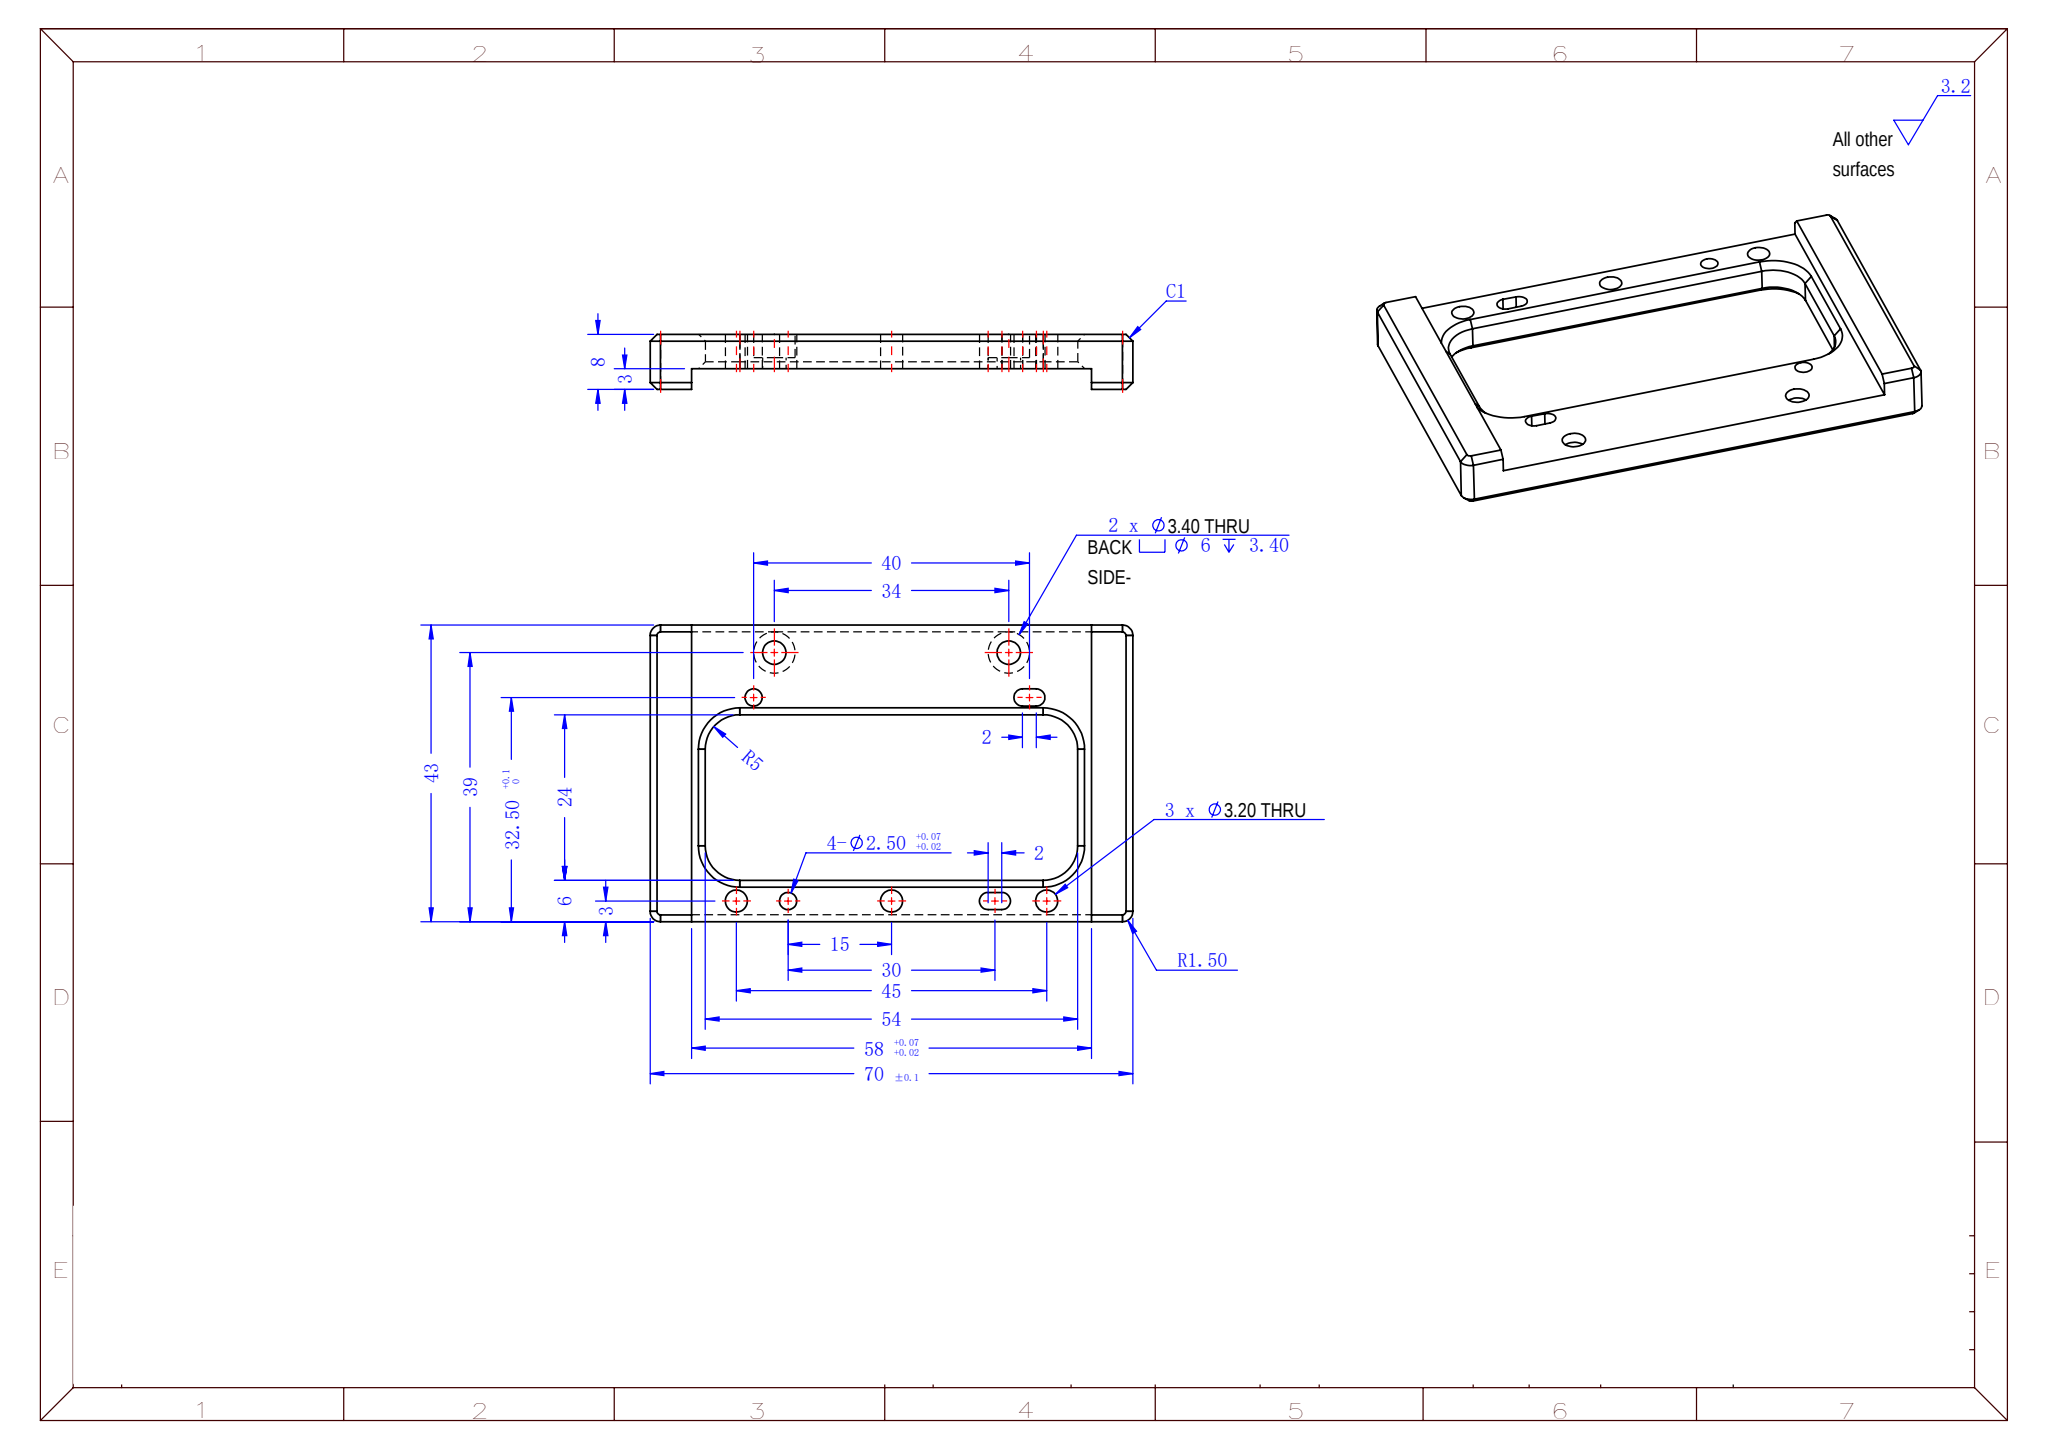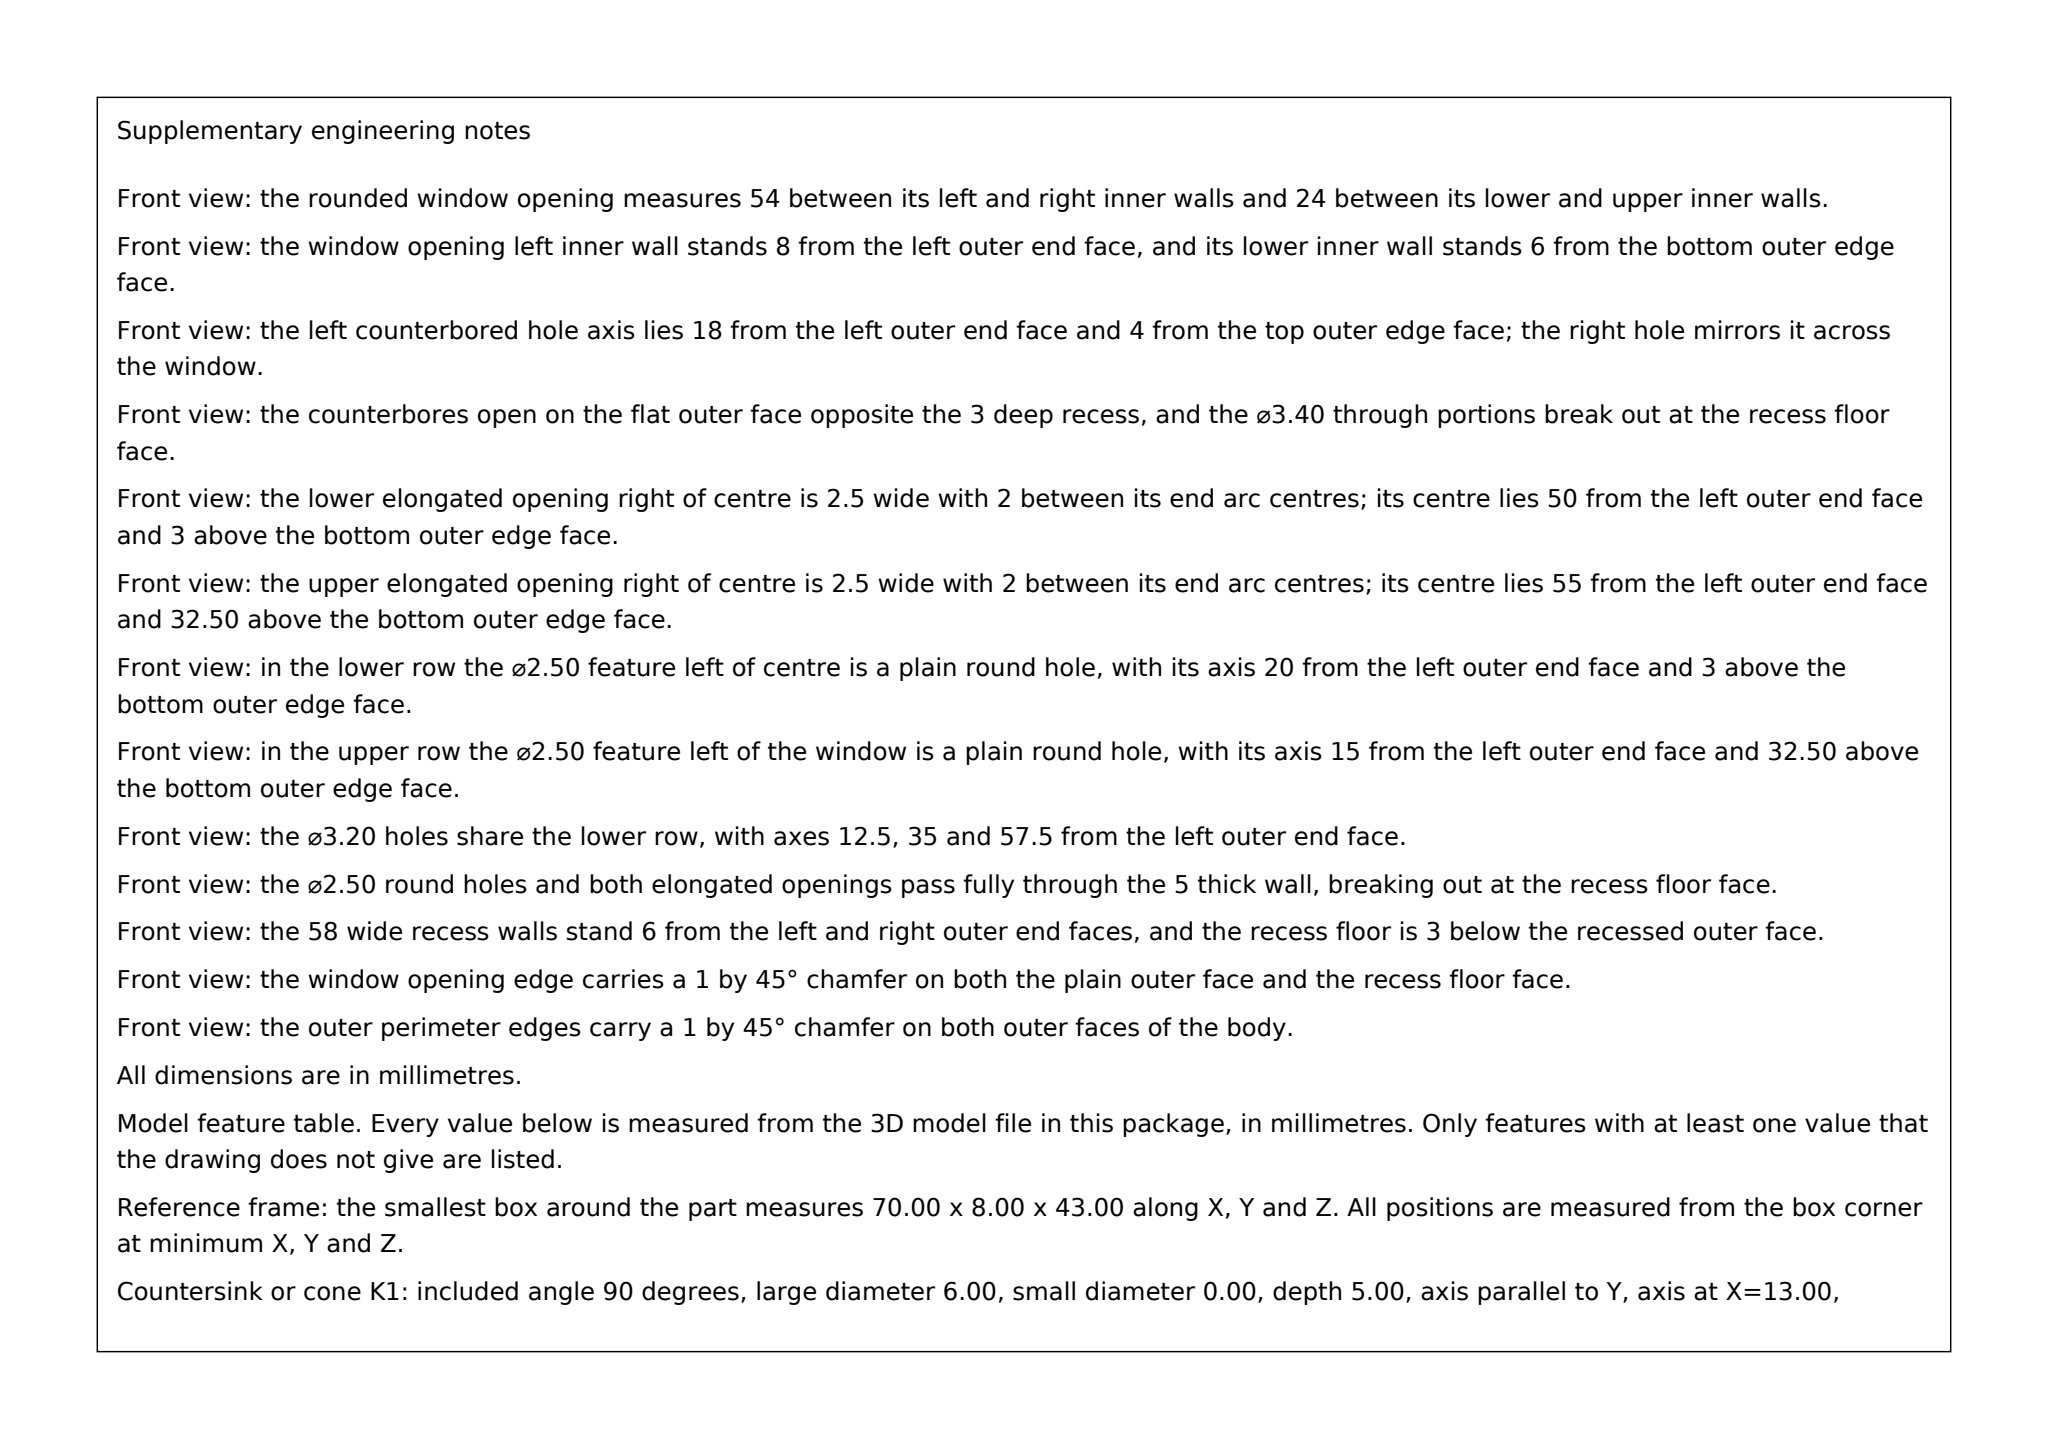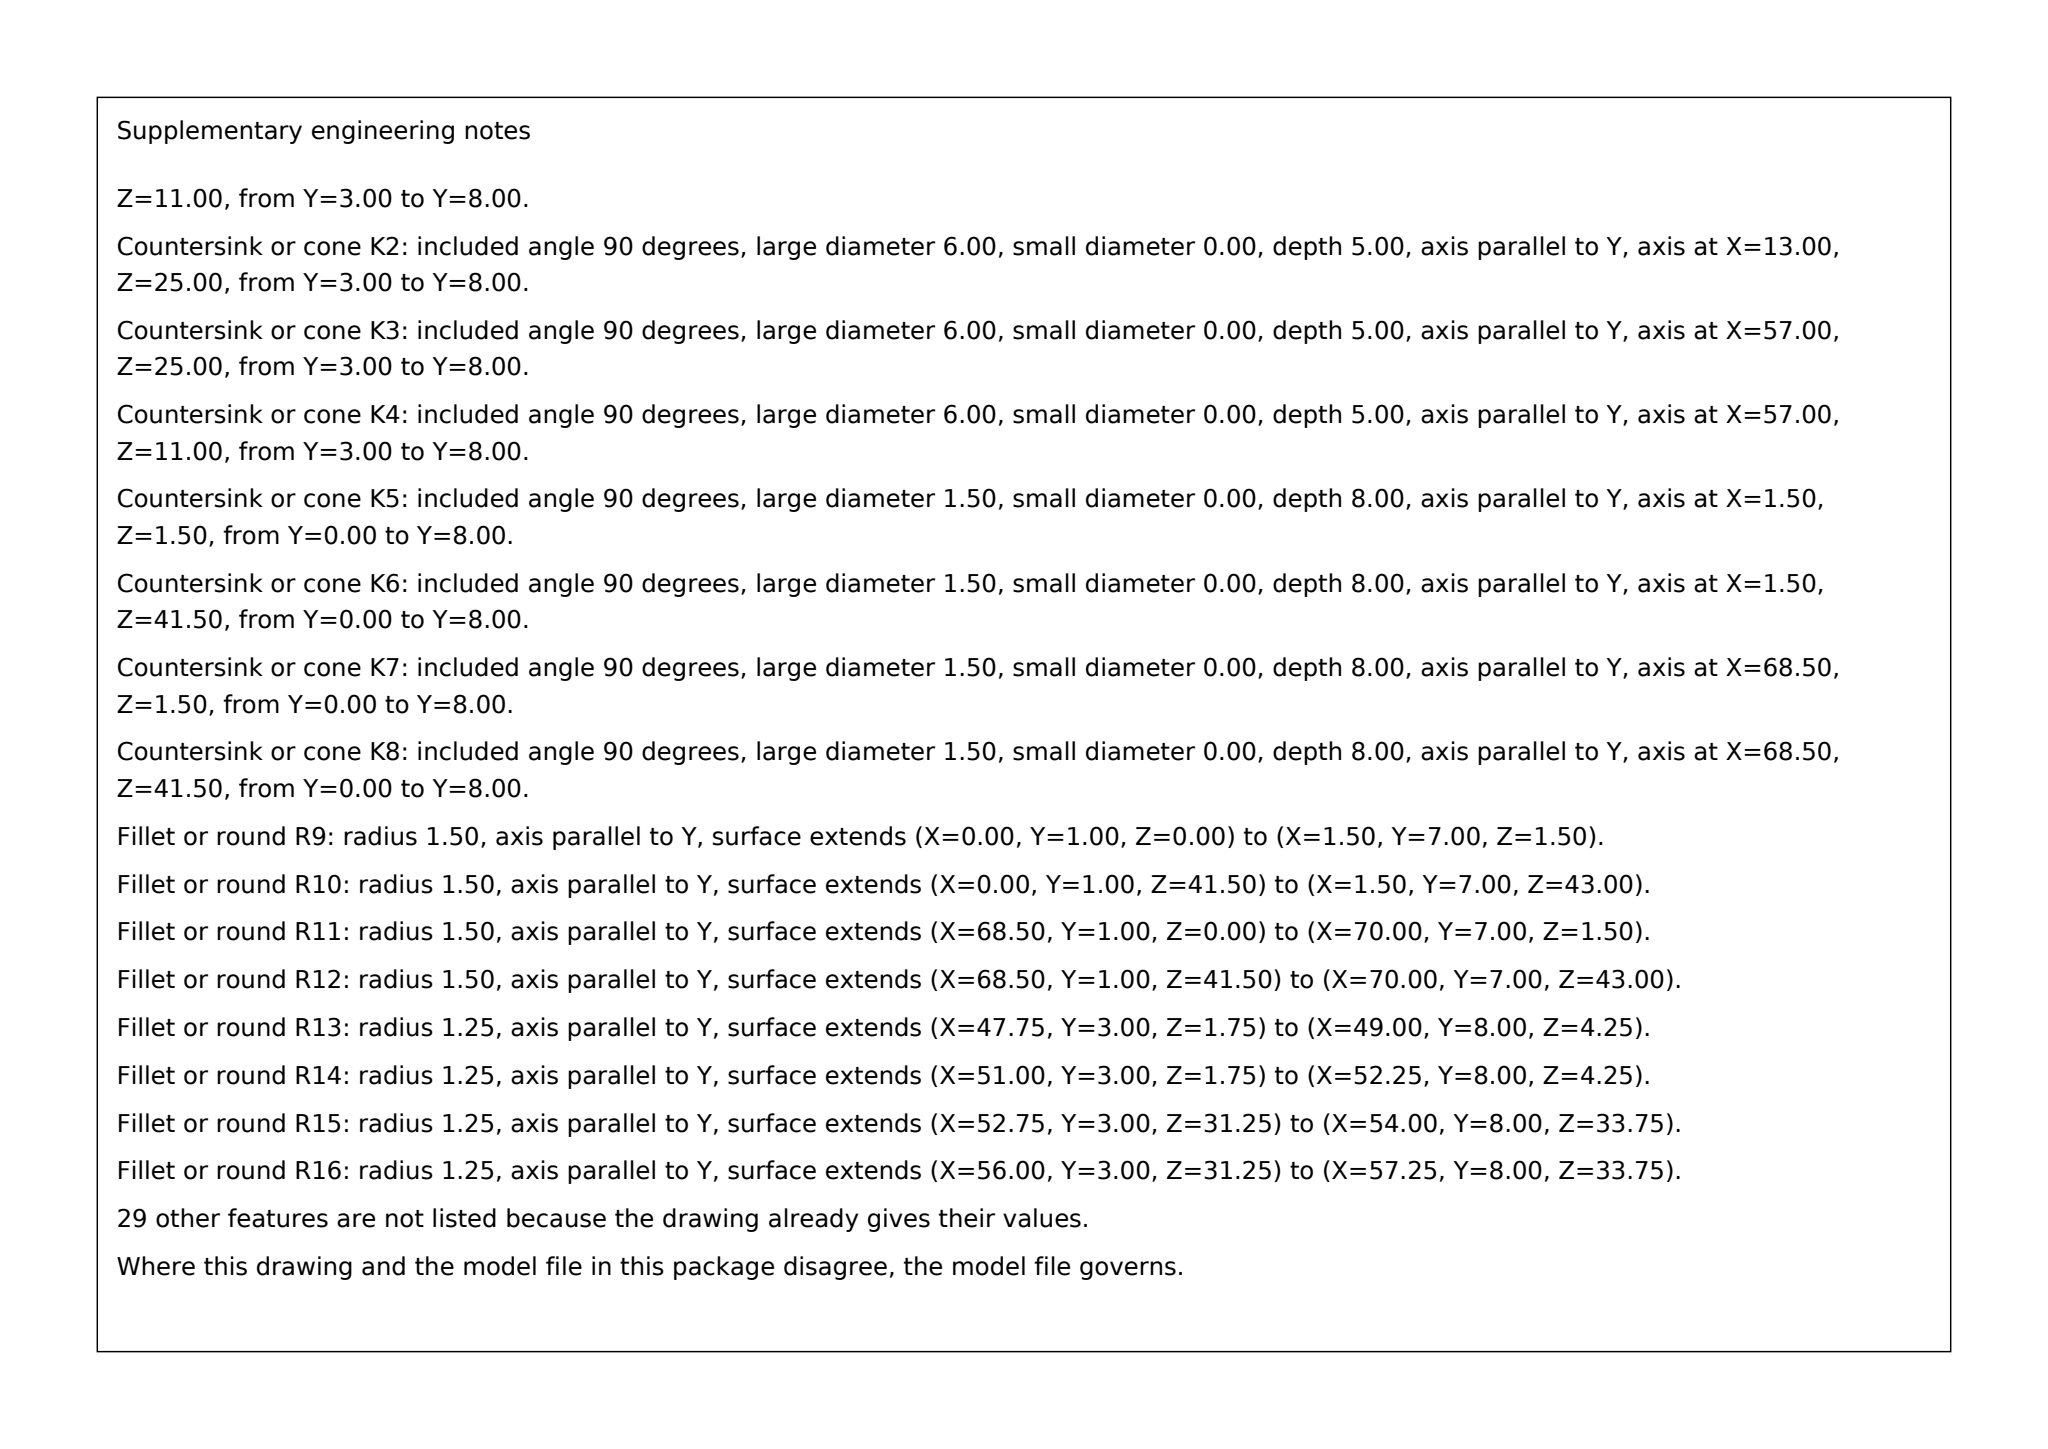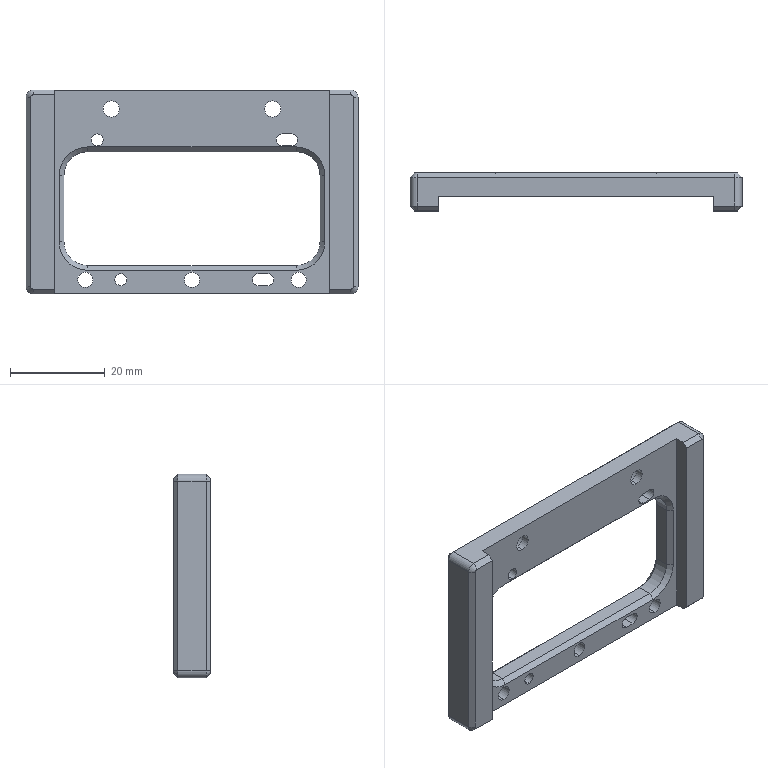Part | SolidWorks | mm | 1 solid | 84 faces | box 70 x 8 x 43 mm | volume 9407 mm3 | plane 38 | cylinder 30 | cone 16 | commonest cylinder face diameters 2.5 x8 3.2 x6 6 x4 3.4 x4 3 x4 10 x4
Drawing notes:
U/SIDE RECESS 58 LG x 3 DP, FULL 43 WD; FOOT 6 WD EA END | from the solid: x-planes 6 & 64 (58 apart), y-plane 3, no z limit planes; bbox z 43
CENTRAL POCKET 54 LG x 24 WD, R5 CORNERS, 8 FR EA END, RAILS FULL HT 8 | from the solid: x-planes 8 & 62 (=54) to ends 0/70, z-planes 6 & 30 (=24), y 0-8
POCKET CL 6 FR LWR EDGE, 13 FR UPPER EDGE IN TOP VIEW | from the solid: z-planes 6 & 30 vs bbox z 0-43
POCKET DP 3.4 FR TOP FACE; FLOOR THK 1.6 | from the solid: y-planes 8 (top), 4.6 (pocket floor), 3 (u/side recess face)
RIM THK 5 ALL ROUND POCKET (TOP FACE AT 8, U/SIDE AT 3) | from the solid: Ø3.2 & Ø2.5 thru holes length 5.0; Ø6 cbore 3.4 + Ø3.4 1.6 = 5
6 x Ø2.50 THRU: UPPER ROW CL 32.5 AT 15/54/56, LWR ROW CL 3 AT 20/49/51 | from the solid: Ø2.5 cyls at x=15/54/56 z=32.5 and x=20/49/51 z=3.0, from LH end x=0